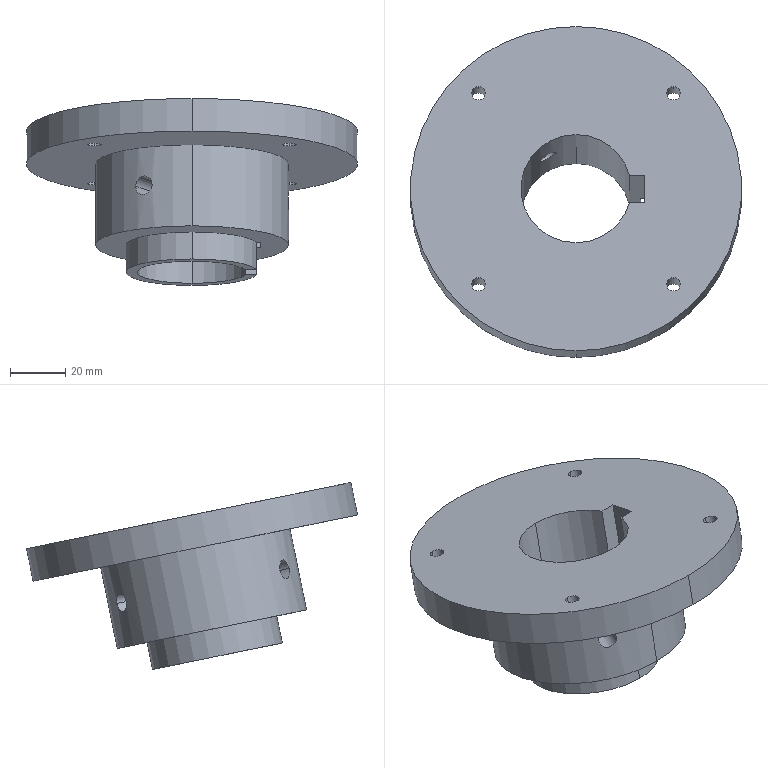Component | SolidWorks | JL001-04-01-007-1 | 1 solid | 31 faces | box 120 x 119.98 x 67.75 mm | volume 198933 mm3 | cylinder 24 | plane 7 | commonest cylinder face diameters 5 x8 6.8 x6 48 x3 40 x3 120 x2 70 x2
build123d program:
from build123d import *

# Parameters (mm, degrees)
SKETCH2_W          = 10
SKETCH2_H          = 10
CUT_EXTRUDE1_DEPTH = 100.519
SKETCH5_W          = 3.4
SKETCH5_H          = 81.962
CIRPATTERN1_COUNT  = 3
M6_TAPPED_HOLE1_D  = 5


with BuildPart() as part:
    # Sketch1 → Revolve1 (revolve)
    with BuildSketch(Plane.XY, mode=Mode.PRIVATE) as revolve1_sk:
        Polygon((0, 20), (0, 24), (-10, 24), (-10, 35), (-40, 35), (-40, 60), (-52, 60), (-52, 20), align=None)
    revolve(revolve1_sk.sketch.rotate(Axis((0, 0, 0), (-1, 0, 0)), 90), axis=Axis((0, 0, 0), (-1, 0, 0)))

    # Sketch2 → Cut-Extrude1 (cut, through all)
    with BuildSketch(Plane.ZY.offset(52)):
        with Locations((0, 20)):
            Rectangle(SKETCH2_W, SKETCH2_H)
    extrude(amount=-CUT_EXTRUDE1_DEPTH, mode=Mode.SUBTRACT)

    # Sketch5 → M8 Tapped Hole2 (revolve, cut)
    with BuildSketch(Plane(origin=(-26, 0, 0), x_dir=(0, 0, -1), z_dir=(1, 0, 0))):
        with Locations((1.7, 40.981)):
            Rectangle(SKETCH5_W, SKETCH5_H)
    m8_tapped_hole2 = revolve(axis=Axis((-26, -6.35, 0), (0, 1, 0)), mode=Mode.SUBTRACT)

    # CirPattern1: M8 Tapped Hole2 ×3 about axis
    cirpattern1_axis = Axis((0, 0, 0), (1, 0, 0))
    for i in range(1, CIRPATTERN1_COUNT):
        add(m8_tapped_hole2.rotate(cirpattern1_axis, i * 360 / CIRPATTERN1_COUNT), mode=Mode.SUBTRACT)

    # M6 Tapped Hole1 (through all)
    with Locations(Plane(origin=(-40, 0, 0), x_dir=(0, 0, -1), z_dir=(1, 0, 0))):
        with Locations((-35.355, 35.355), (35.355, 35.355), (35.355, -35.355), (-35.355, -35.355)):
            Hole(M6_TAPPED_HOLE1_D / 2)


solid = part.part

# Placed as in the assembly
solid = solid.moved(Location((0, 195.722, 129.474), (78.465, 0.0003261, -90)))